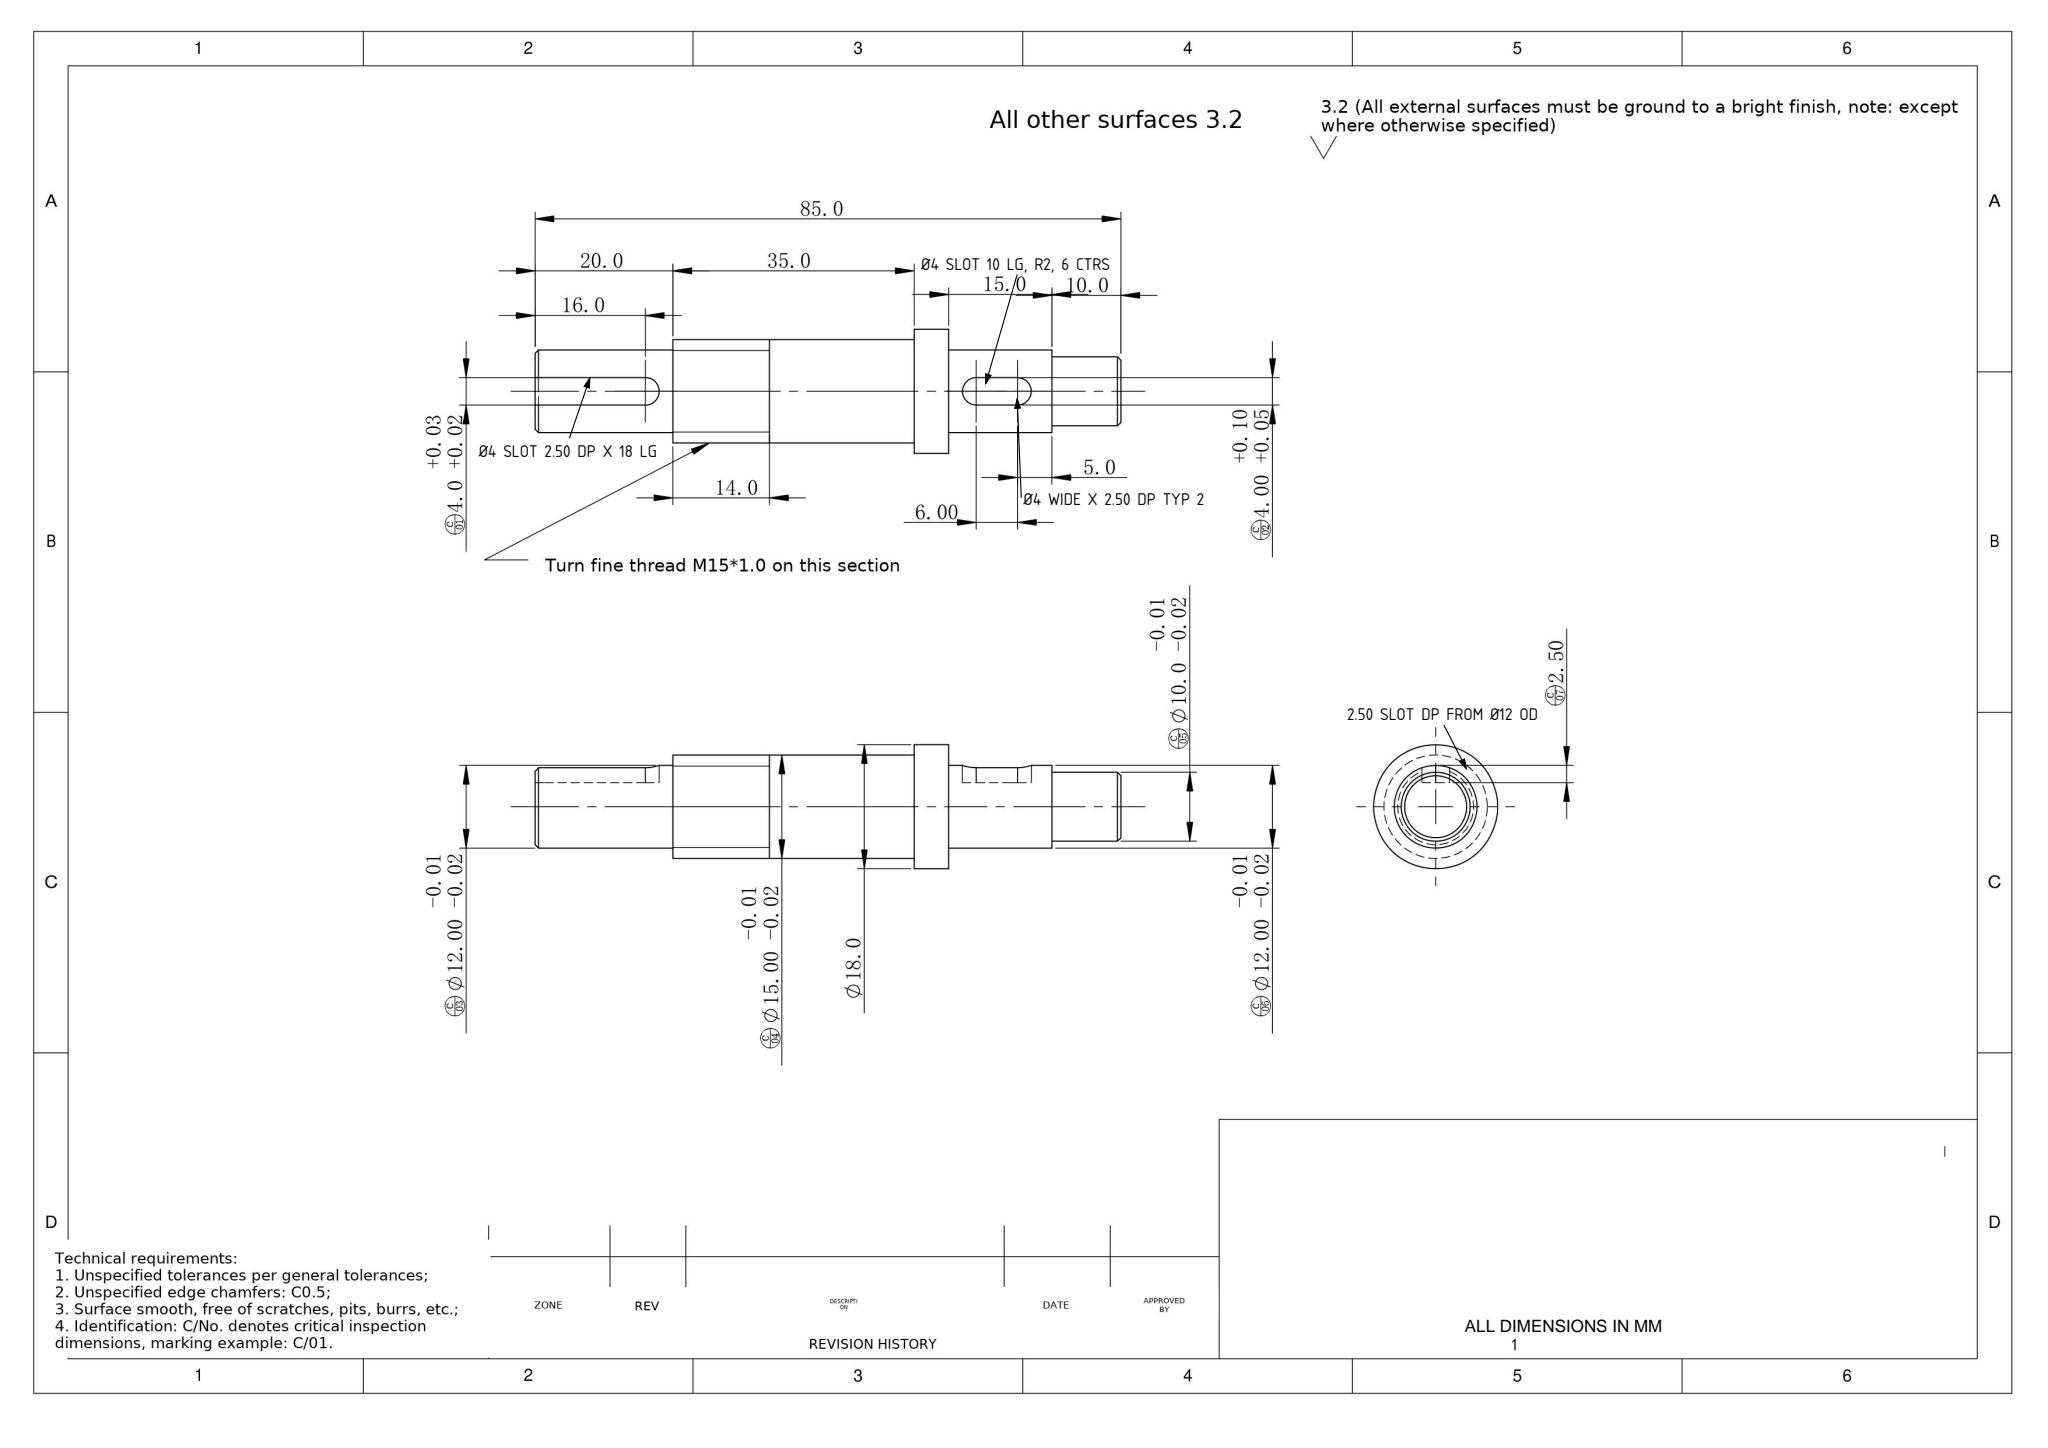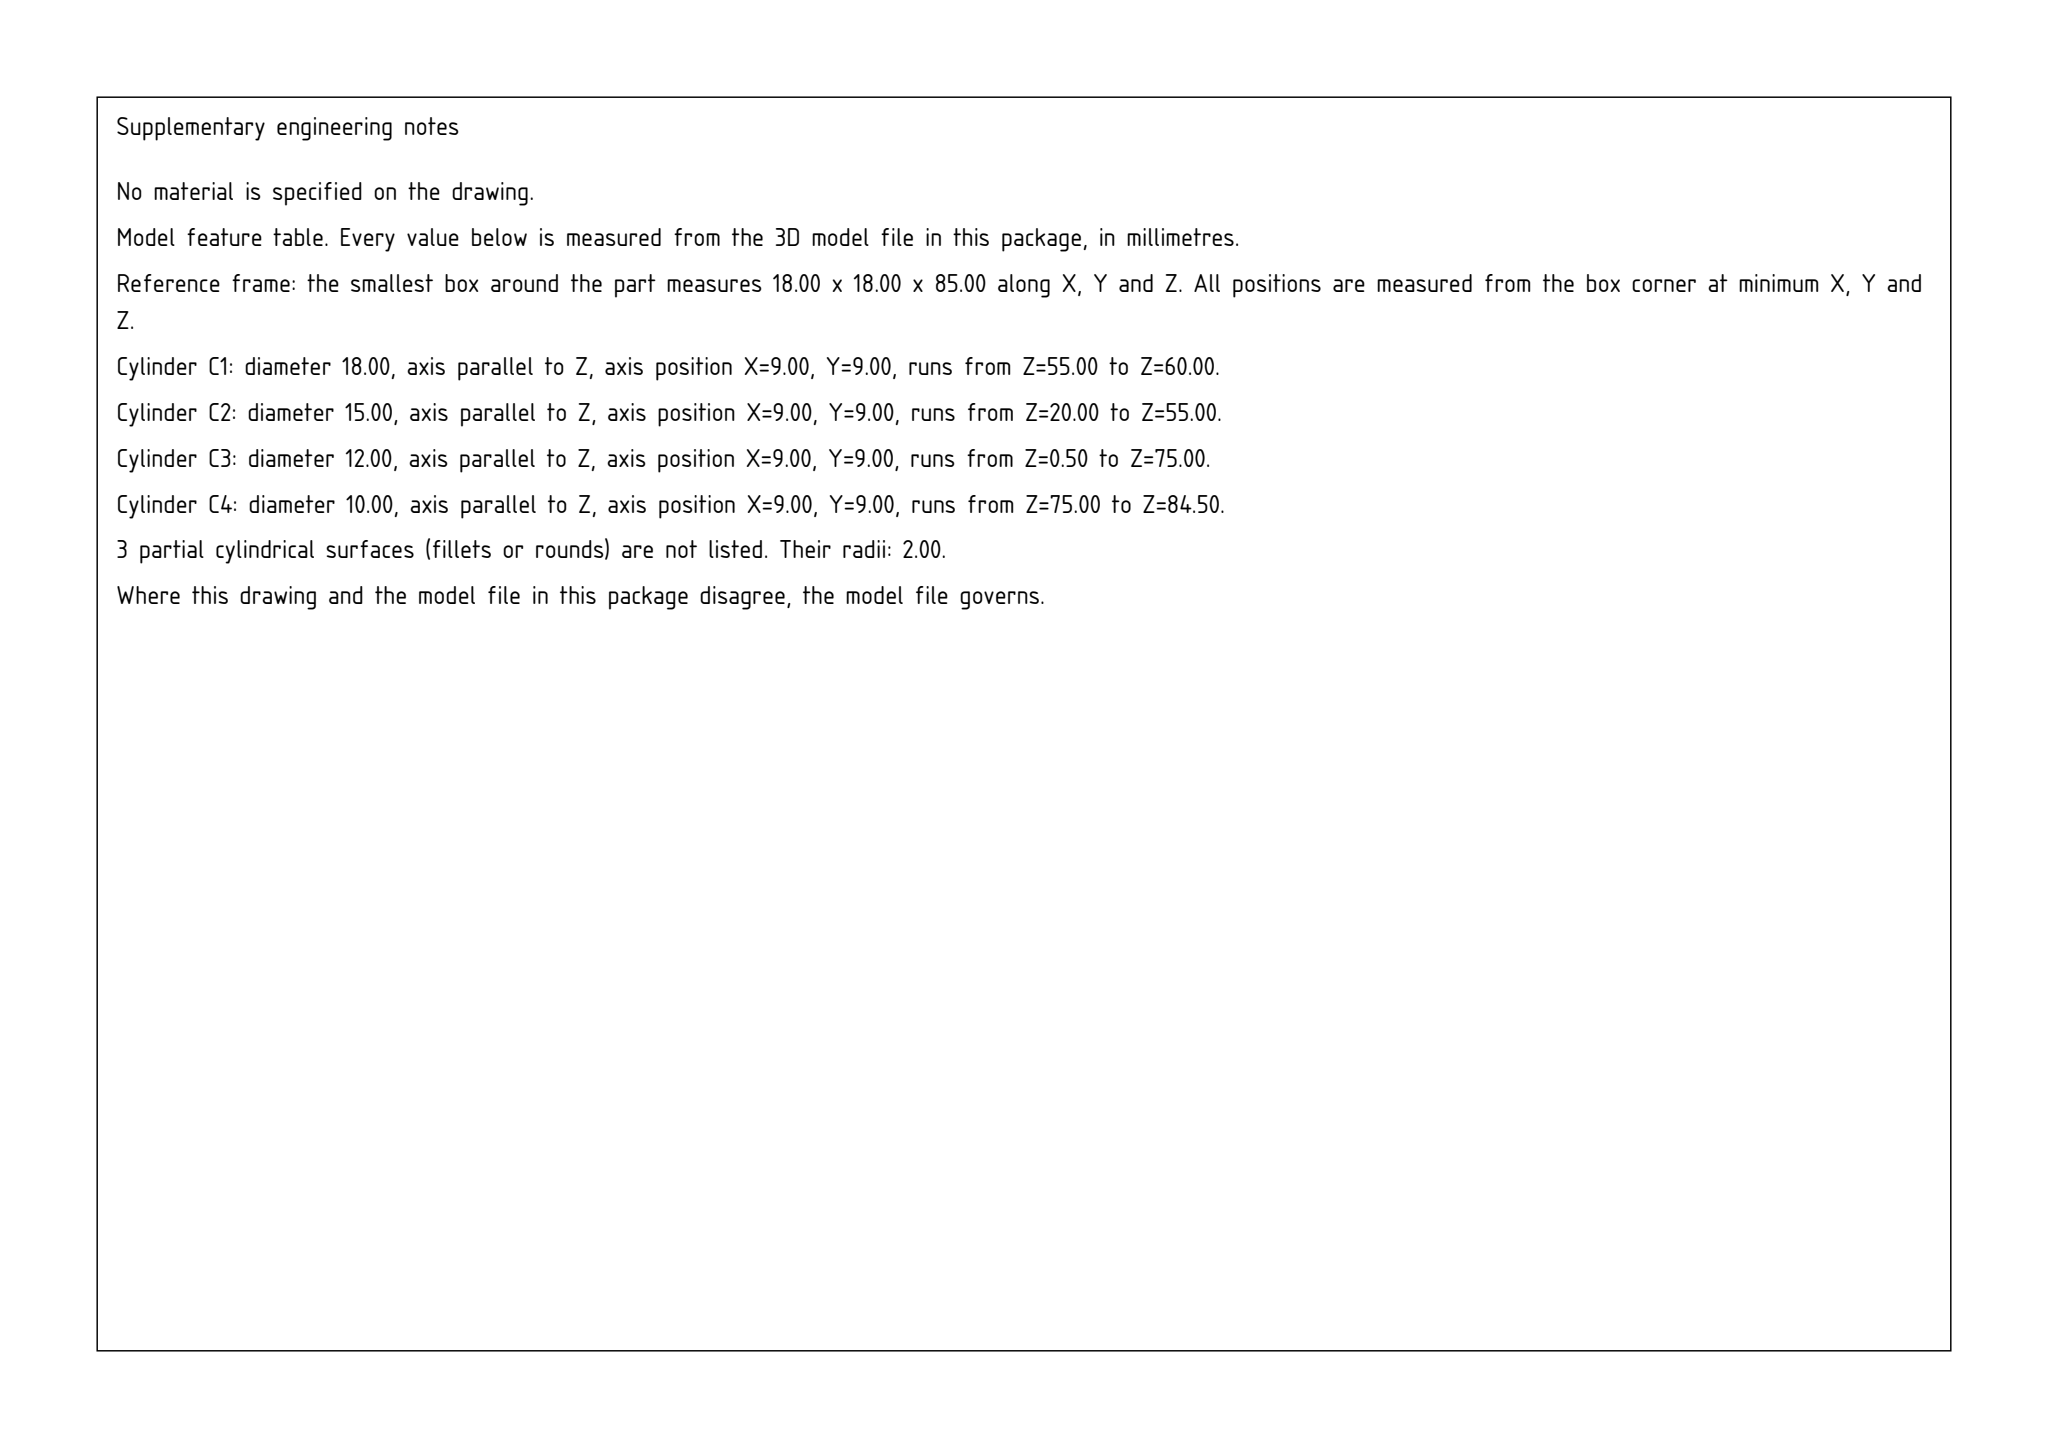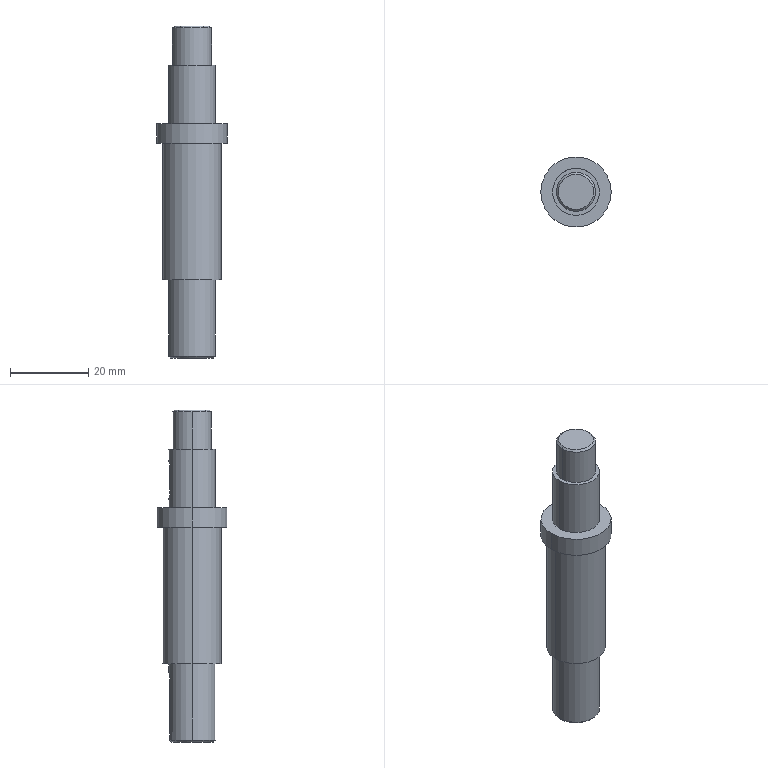Part | SolidWorks | mm | 1 solid | 33 faces | box 18 x 18 x 85 mm | volume 11938 mm3 | cylinder 16 | plane 12 | cone 5 | commonest cylinder face diameters 4 x6 12 x4 10 x2 18 x2 15 x2
Drawing notes:
RH SLOT ON Ø12: Ø4 WIDE x 2.50 DP - DEPTH TYP BOTH SLOTS | from the solid: Ø4 y-axis cyls at z=64 & z=70 (x=9), len 2.5 each; flat plane y=12.5 = 2.50 below Ø12 OD top (y=15); same 2.5 depth as Ø4 slot at z=16
Ø4 LH SLOT: 2.5 DEEP FROM Ø12 OD, OPEN AT END FACE, 18 LG | from the solid: Slot walls x=7 & x=11 (4 wide), floor plane y=12.5 vs Ø12 OD top y=15.0 => 2.5 deep; floor extent z=0 to 18 with R2 end arc (dia 4, axis y) at z=16; open at z=0 end face
Ø4.00 RH SLOT: 2.5 DEEP FROM Ø12 OD, 10 LG, R2 ENDS, 6 CTRS | from the solid: Floor plane y=12.5 (OD top y=15.0 => 2.5 deep) extent z=62-72 on Ø12 (z=60-75); dia-4 y-axis end arcs at z=64 and z=70 (6 apart), overall 10 long
2.50 IN END VIEW = SLOT DEPTH FROM Ø12 OD, TYP BOTH SLOTS | from the solid: Only 2.5 dimension in model: Ø12 OD top y=15.0 minus slot floor y=12.5; same floor height for slot z=0-18 and slot z=62-72